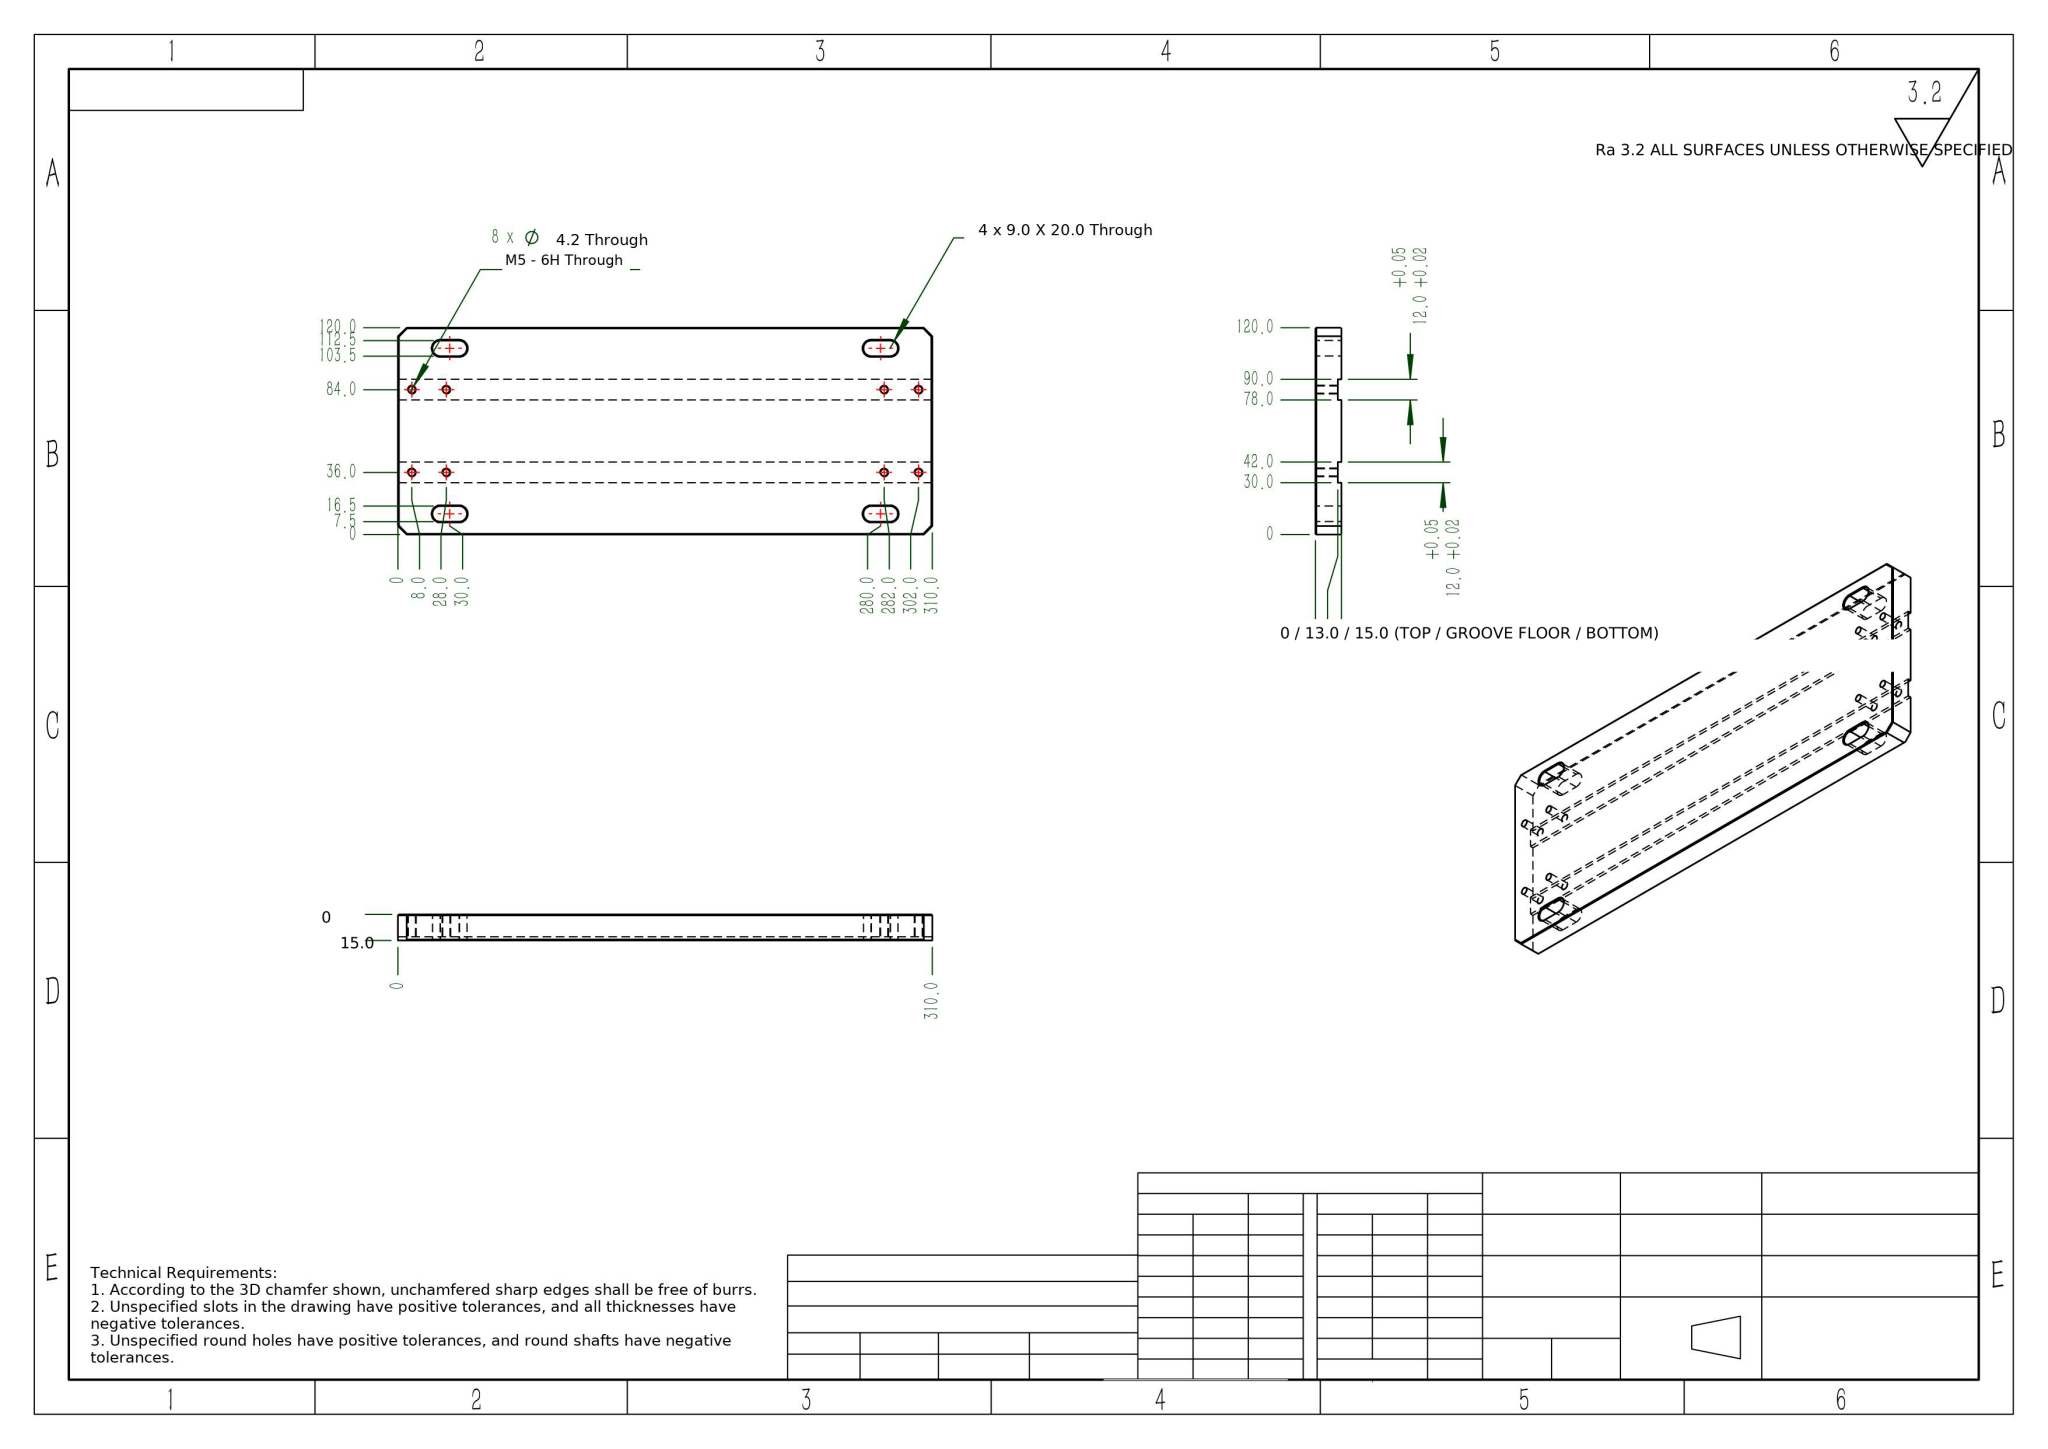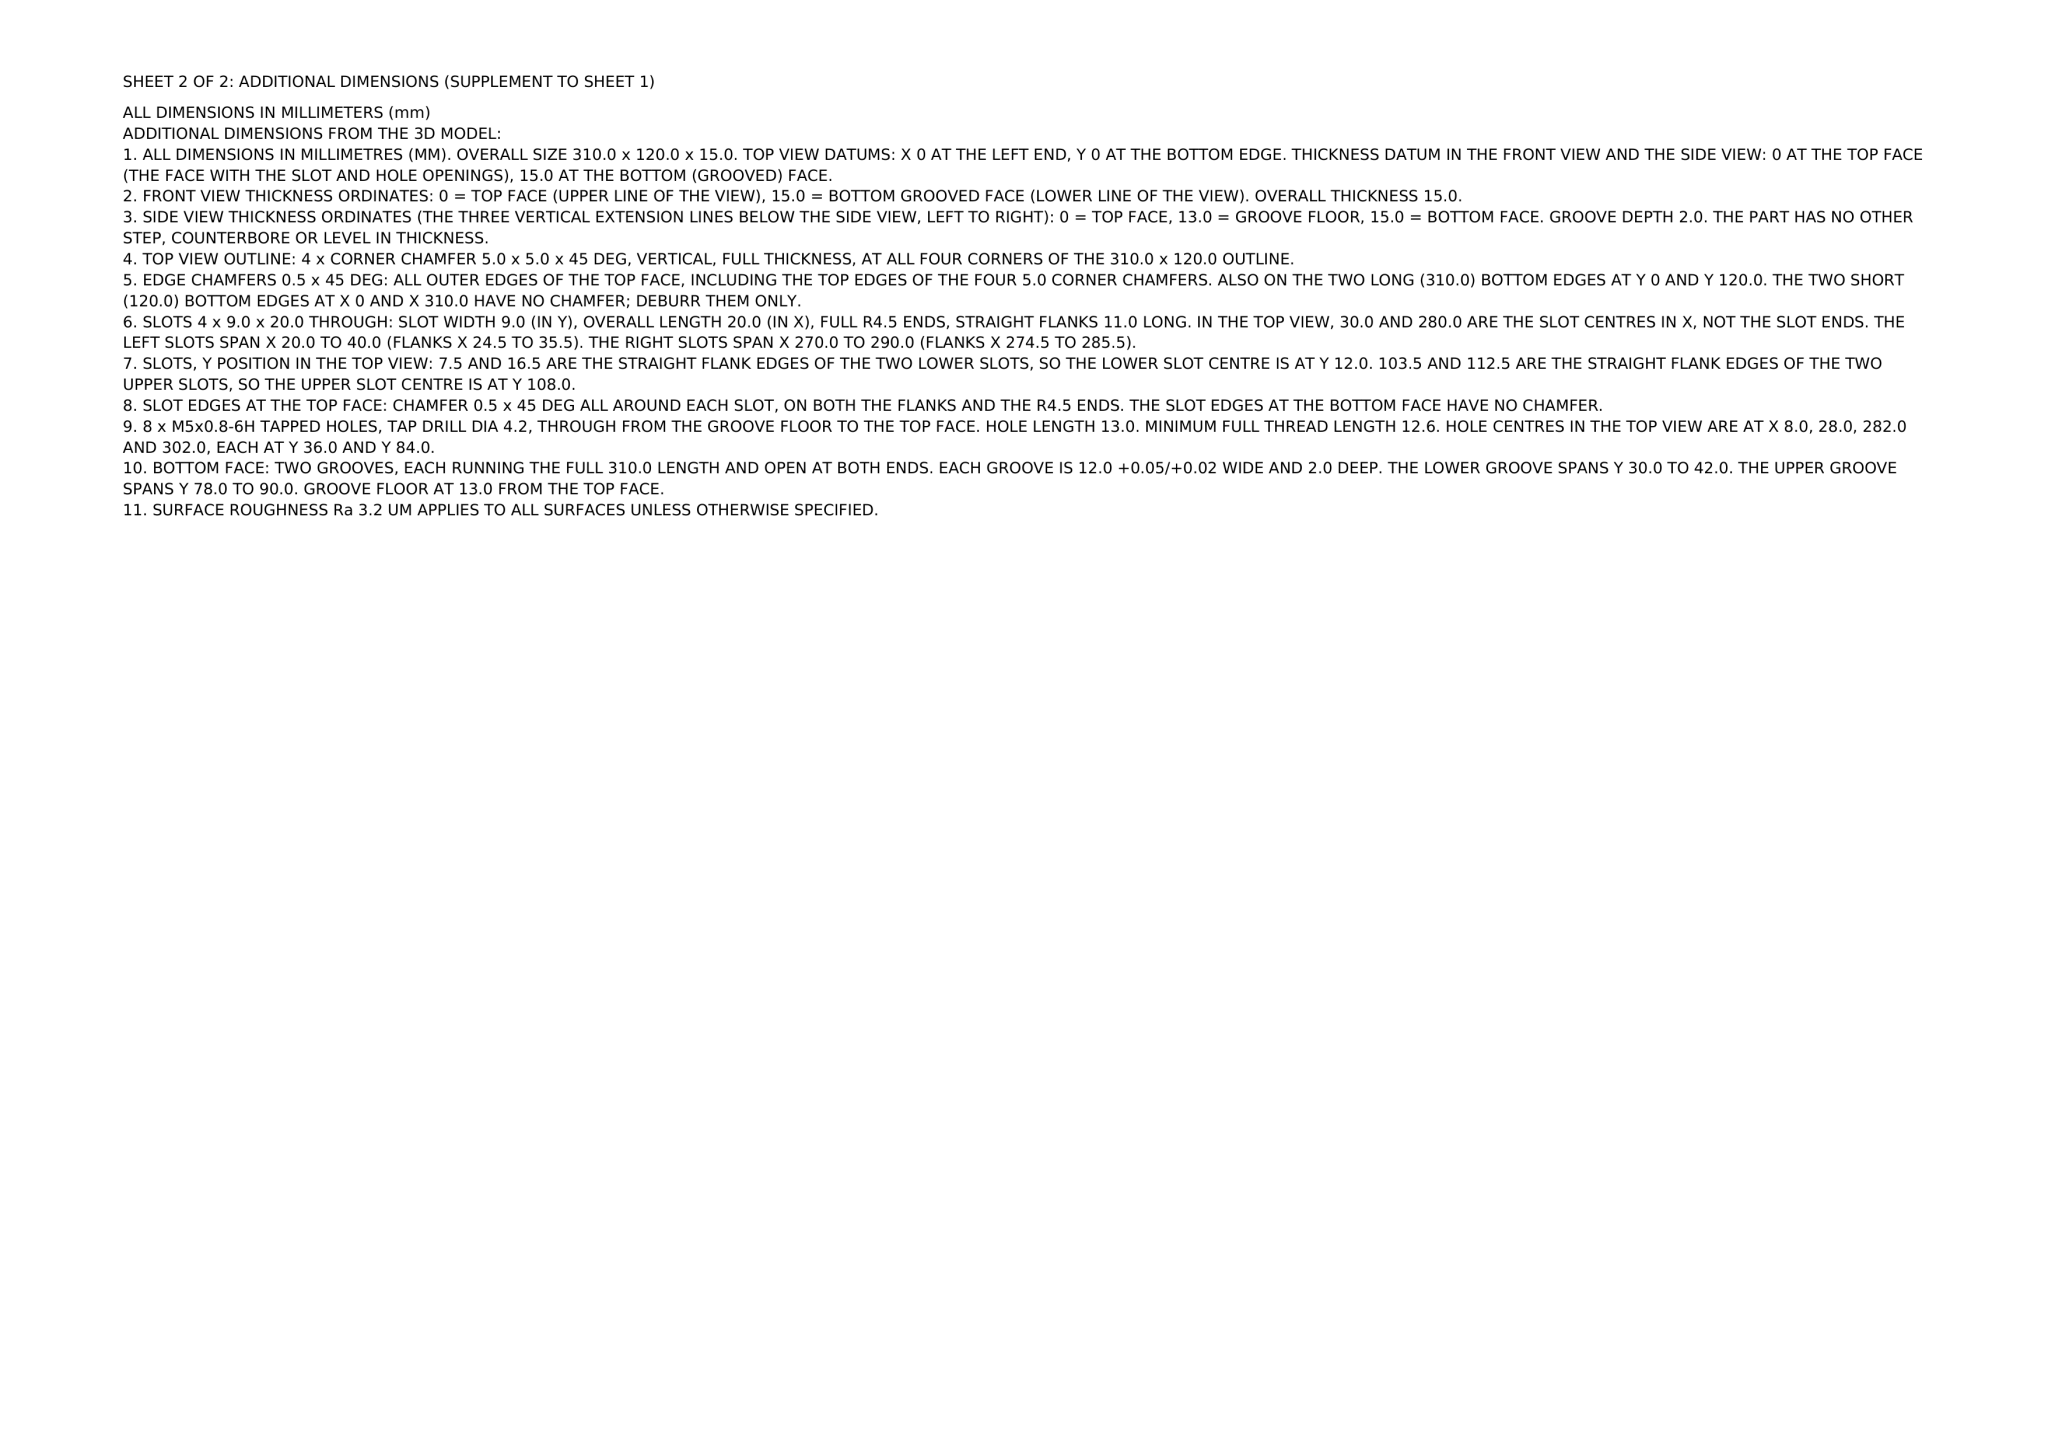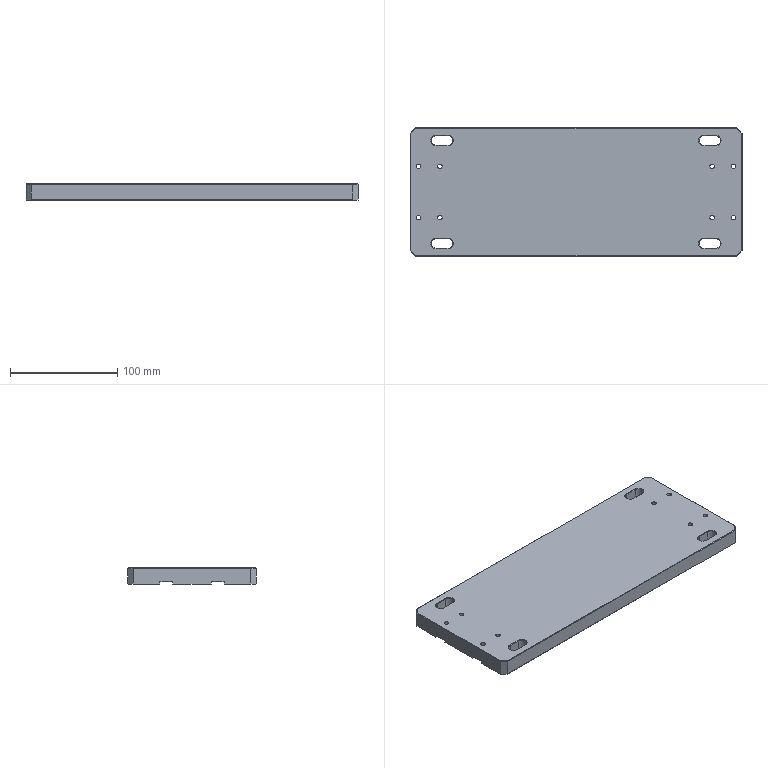Part | NX | mm | 1 solid | 84 faces | box 310 x 120 x 15 mm | volume 530965 mm3 | plane 44 | cylinder 28 | cone 12 | commonest cylinder face diameters 4.2 x16 9 x12